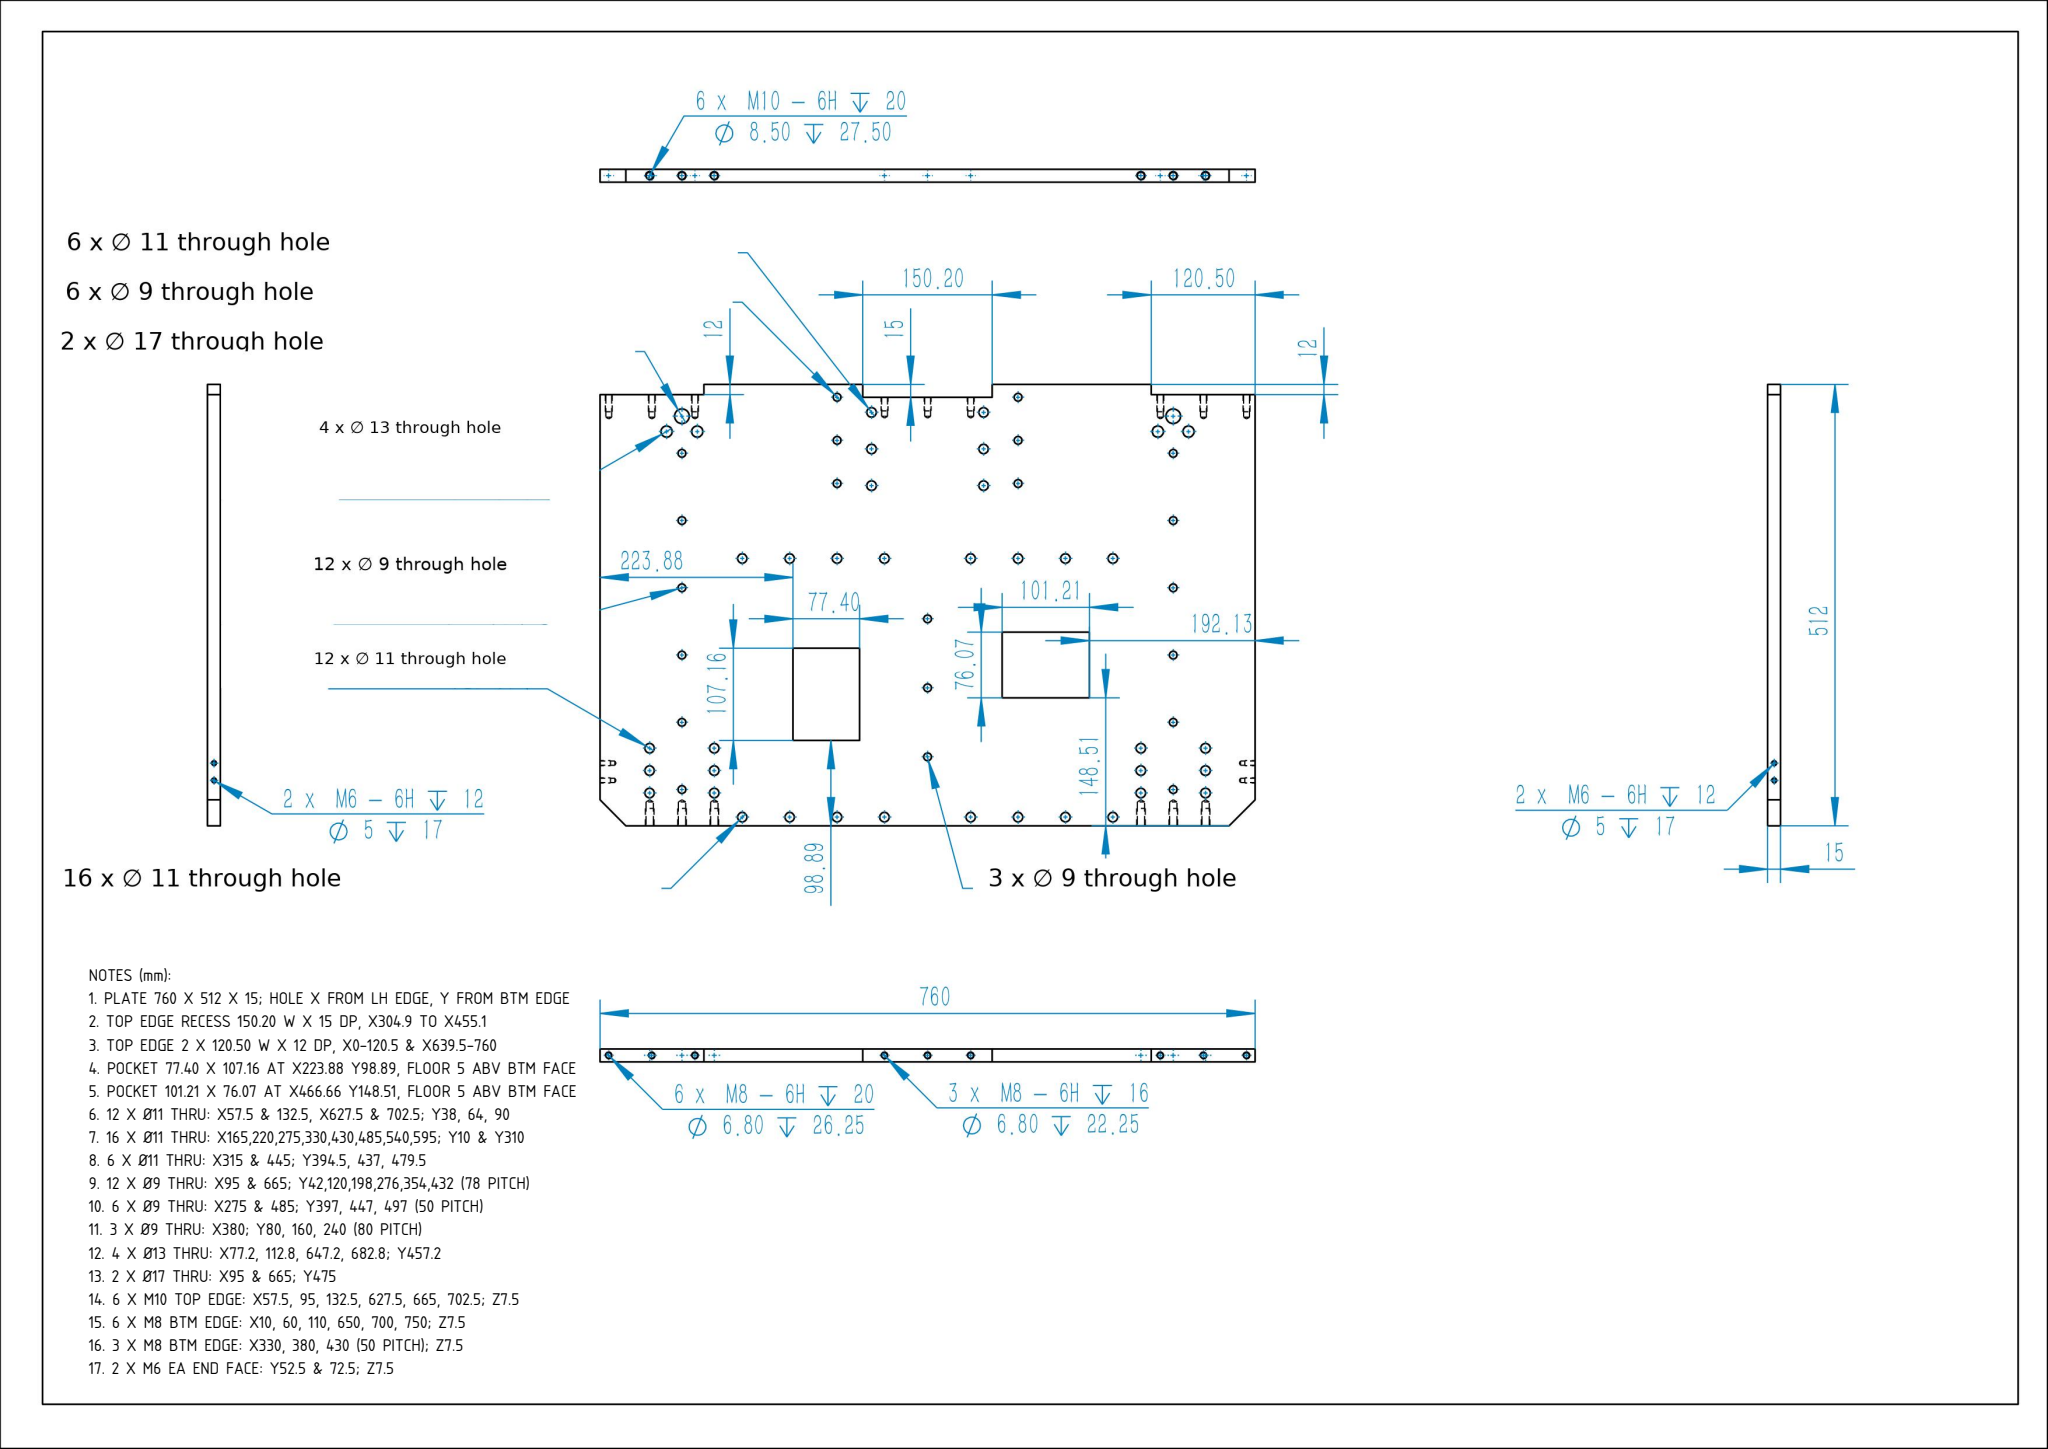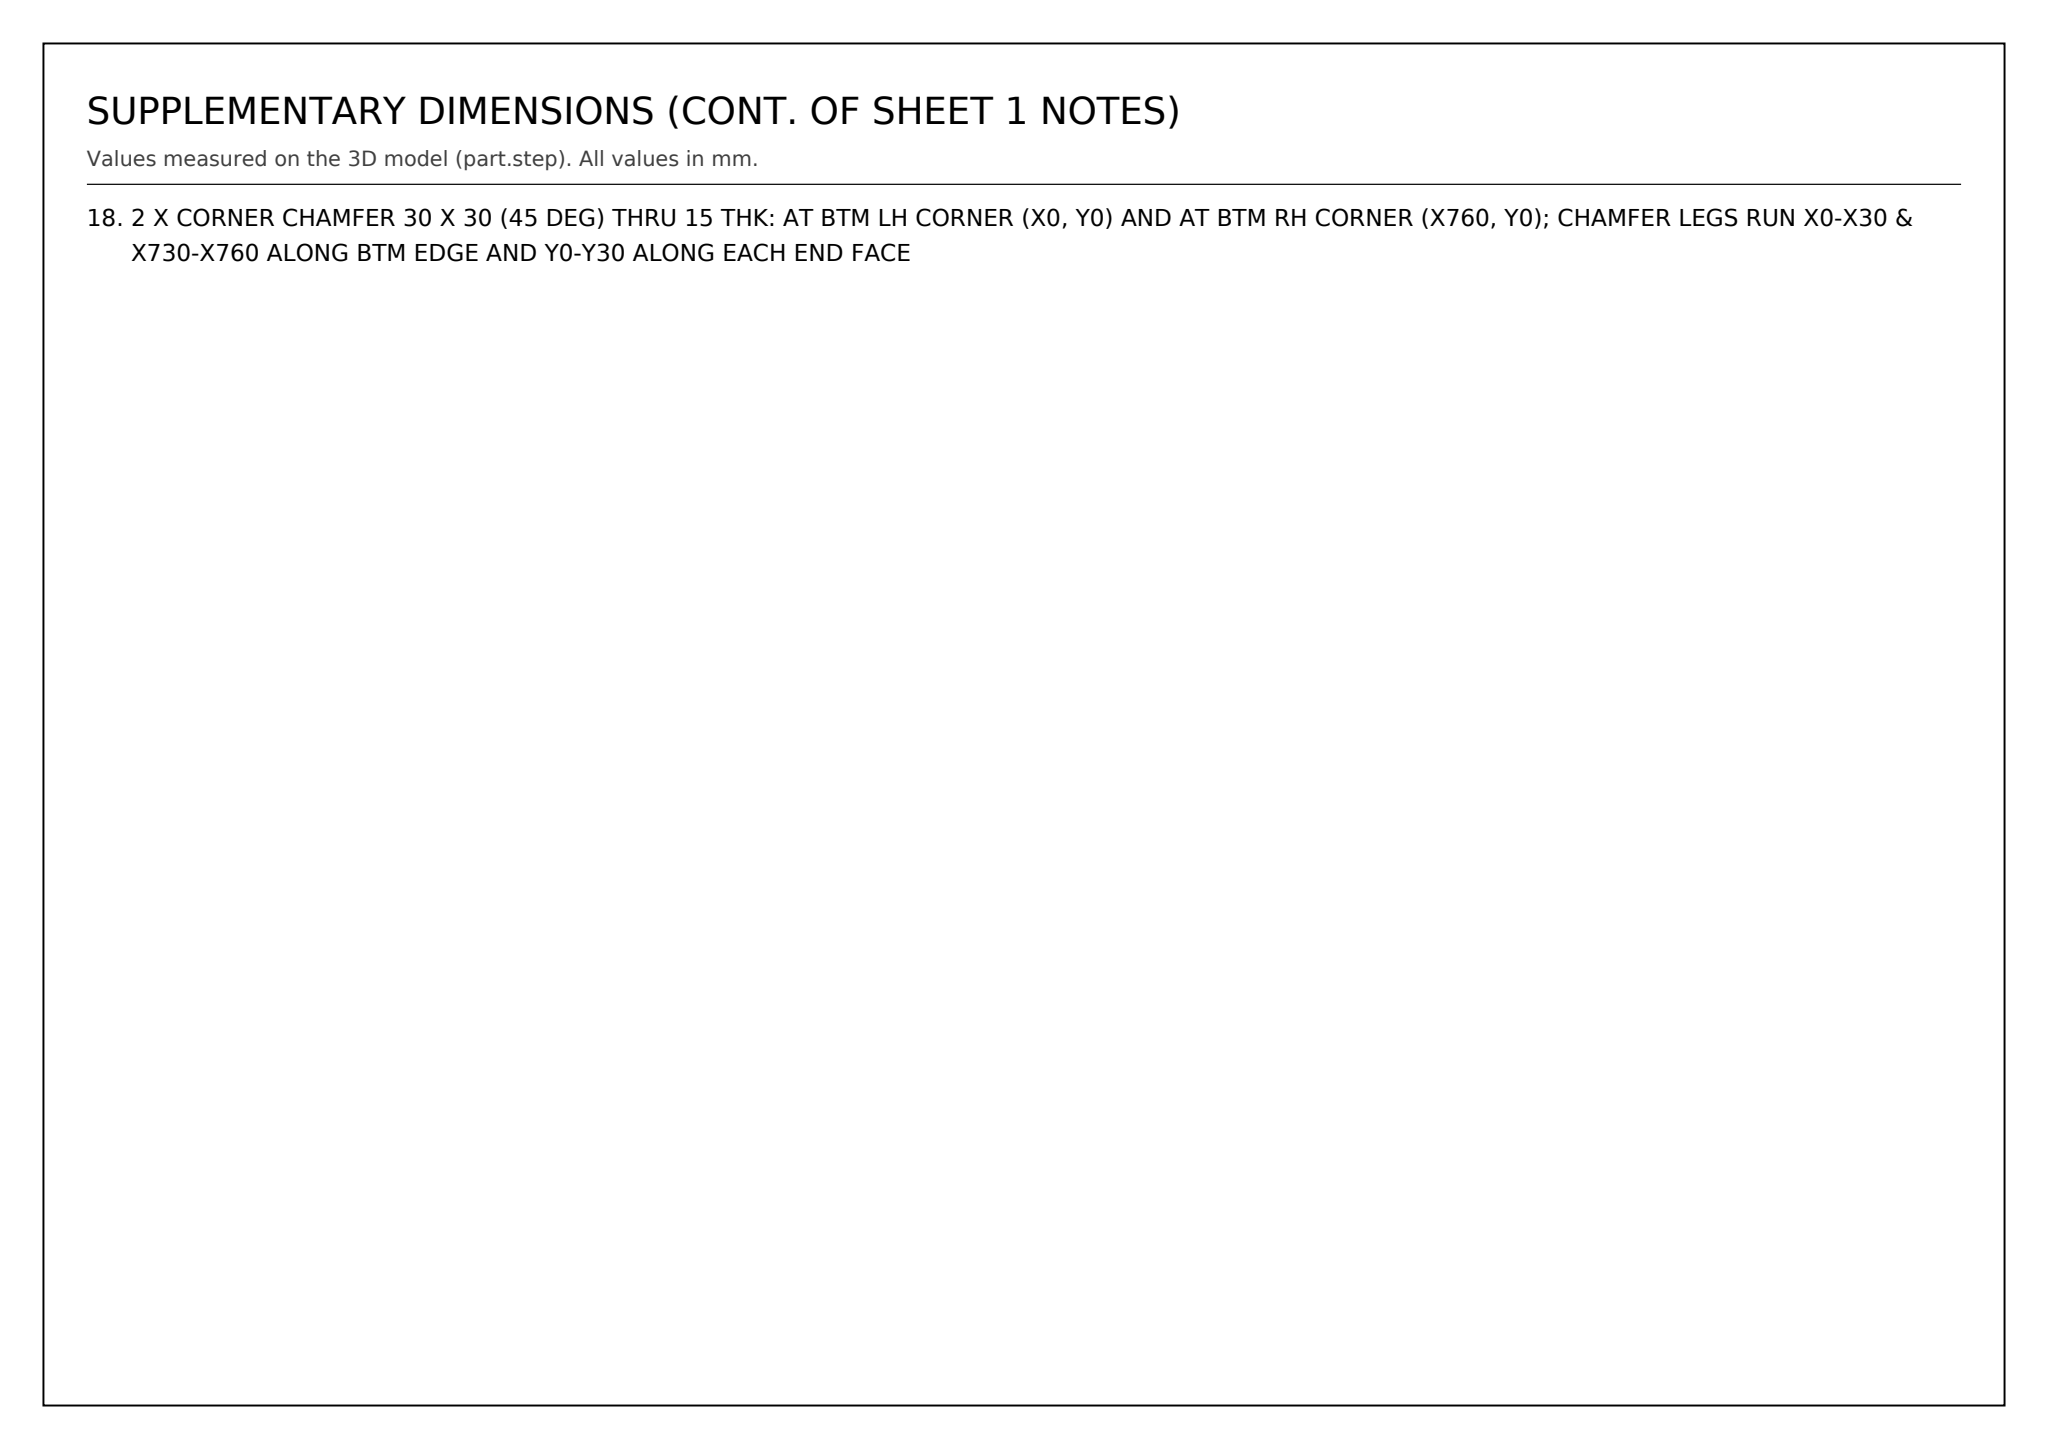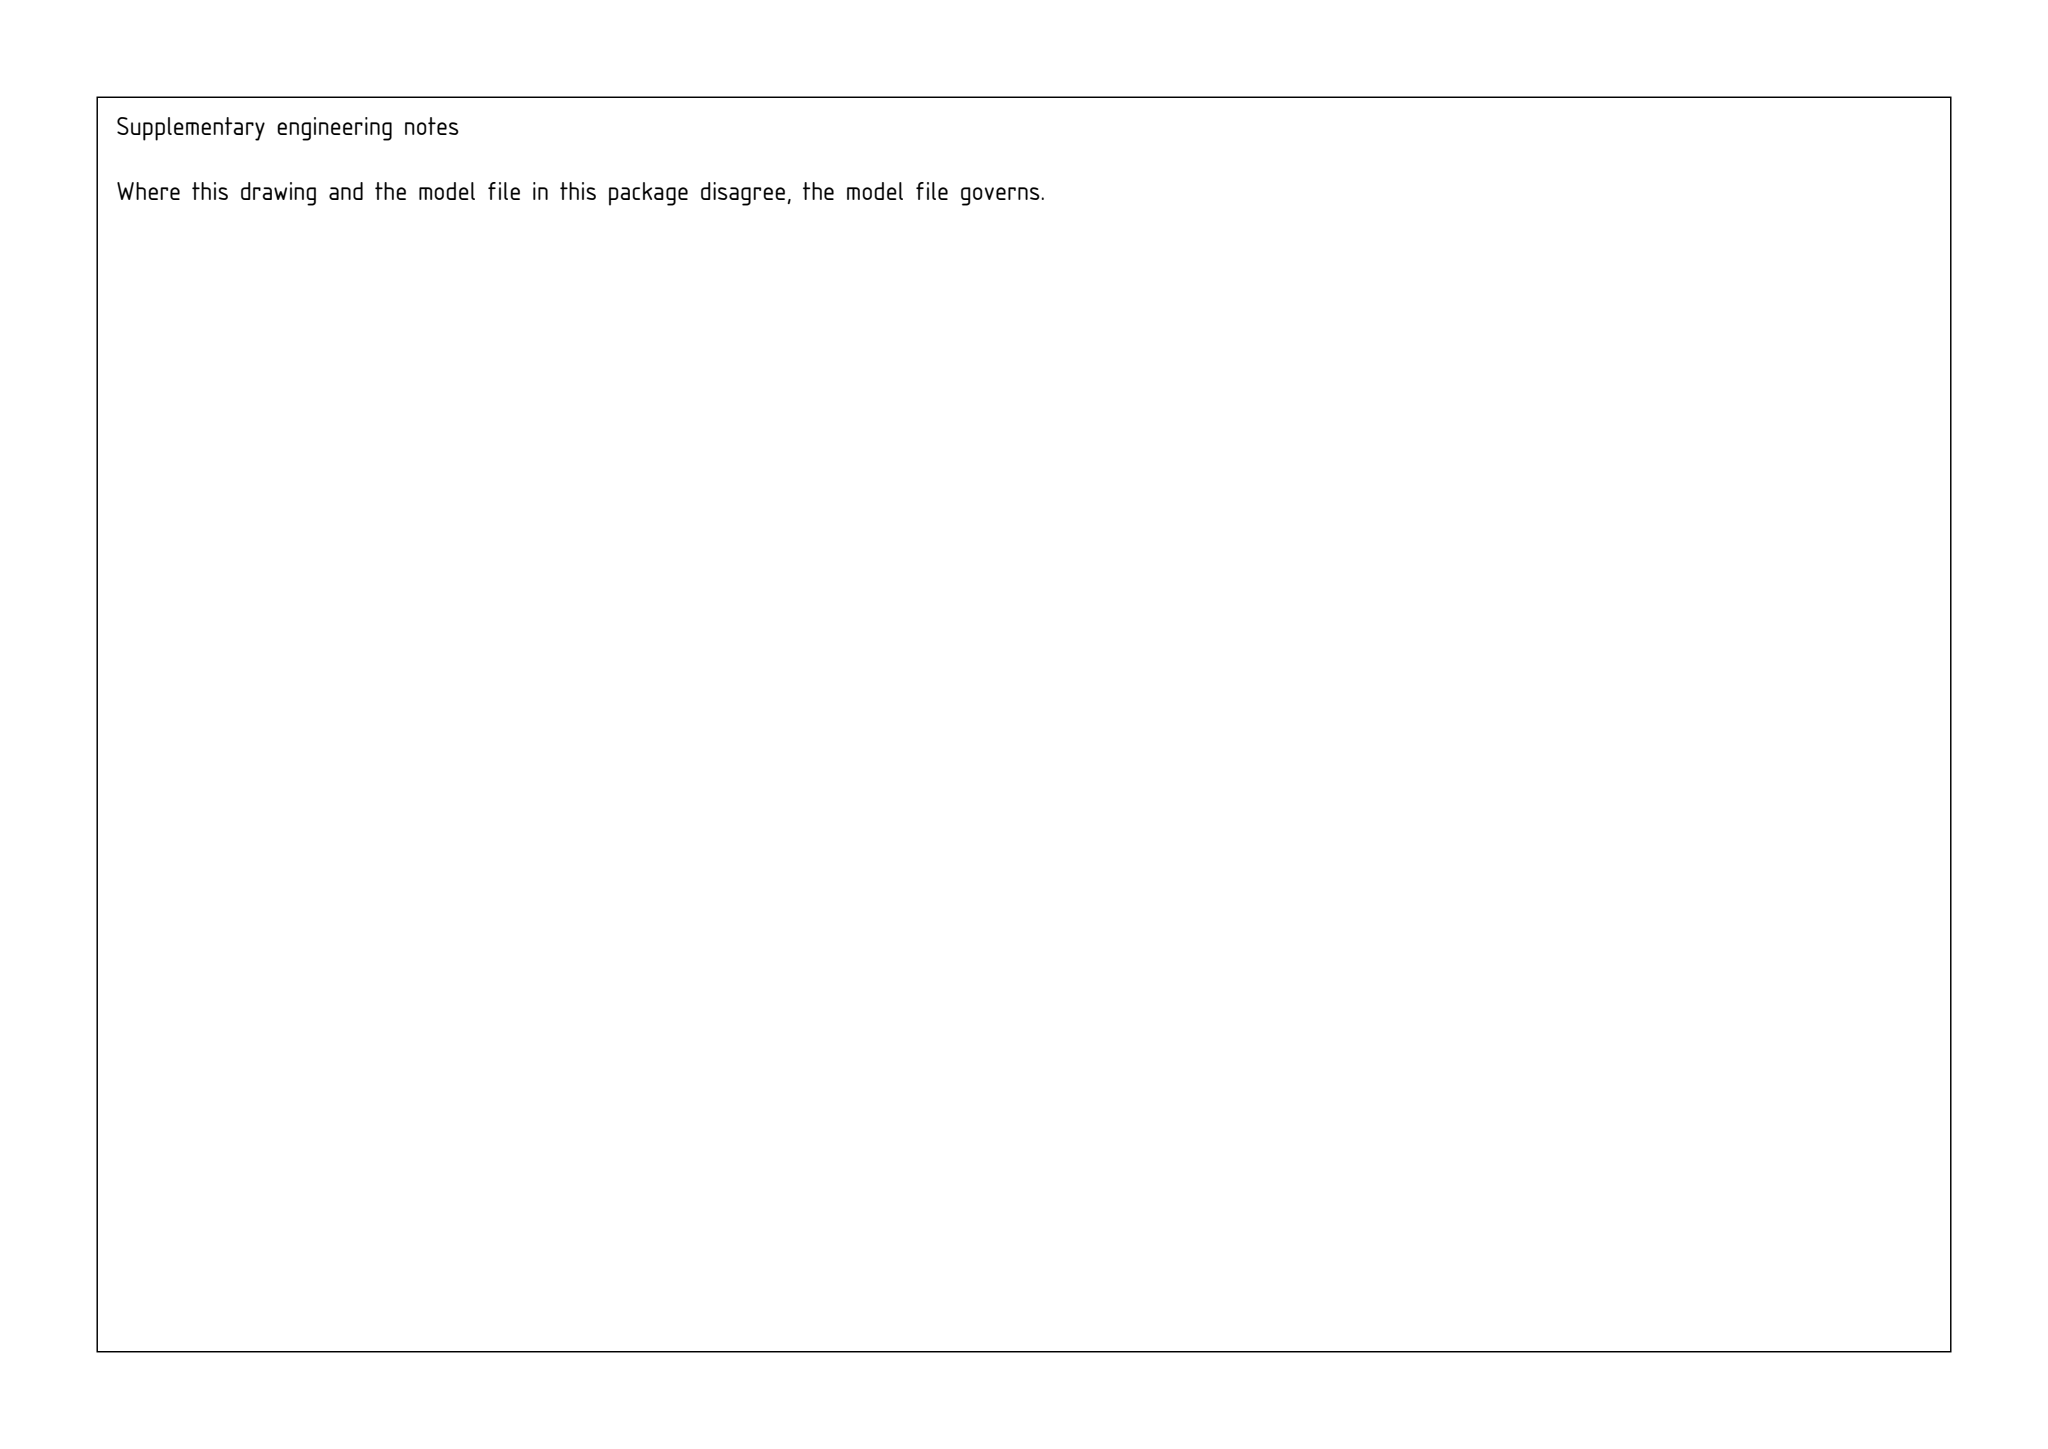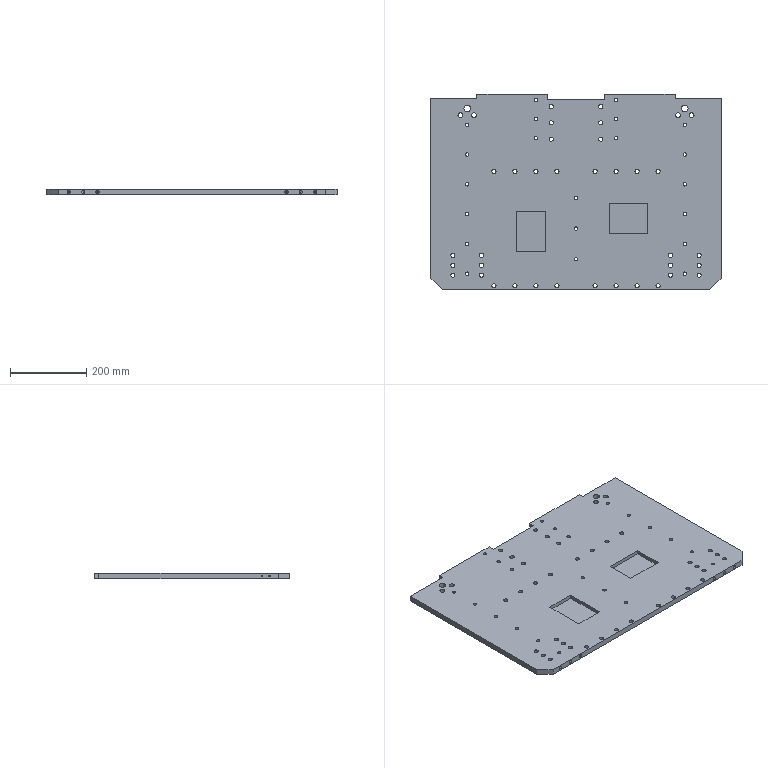Part | SolidWorks | mm | 1 solid | 224 faces | box 760 x 512 x 15 mm | volume 5483517 mm3 | cylinder 160 | cone 38 | plane 26 | commonest cylinder face diameters 11 x68 9 x42 6.8 x18 8.5 x12 5 x8 13 x8 17 x4
Drawing notes:
PLATE 760 X 512 X 15; HOLE X FROM LH EDGE, Y FROM BTM EDGE | from the solid: bbox_xyz [760,512,15], positions from min corner of bbox
TOP EDGE RECESS 150.20 W X 15 DP, X304.9 TO X455.1 | from the solid: x planes 304.9/455.1, y plane 497 vs 512 edge
TOP EDGE 2 X 120.50 W X 12 DP, X0-120.5 & X639.5-760 | from the solid: x planes 120.5/639.5, y planes 500 (2 faces) vs 512
POCKET 77.40 X 107.16 AT X223.88 Y98.89, FLOOR 5 ABV BTM FACE | from the solid: x planes 223.88/301.28, y planes 98.89/206.06, z plane 5
POCKET 101.21 X 76.07 AT X466.66 Y148.51, FLOOR 5 ABV BTM FACE | from the solid: x planes 466.66/567.87, y planes 148.51/224.58, z plane 5
12 X Ø11 THRU: X57.5 & 132.5, X627.5 & 702.5; Y38, 64, 90 | from the solid: Ø11 cyls at (57.5/132.5/627.5/702.5, 38/64/90), L=15 thru
16 X Ø11 THRU: X165,220,275,330,430,485,540,595; Y10 & Y310 | from the solid: Ø11 cyls at those X with y=10 and y=310, L=15 thru
6 X Ø11 THRU: X315 & 445; Y394.5, 437, 479.5 | from the solid: Ø11 cyls (315/445, 394.5/437/479.5), L=15 thru
12 X Ø9 THRU: X95 & 665; Y42,120,198,276,354,432 (78 PITCH) | from the solid: Ø9 cyls at x=95 & 665, y=42..432 step 78, L=15 thru
6 X Ø9 THRU: X275 & 485; Y397, 447, 497 (50 PITCH) | from the solid: Ø9 cyls at x=275 & 485, y=397/447/497, L=15 thru
3 X Ø9 THRU: X380; Y80, 160, 240 (80 PITCH) | from the solid: Ø9 cyls at x=380, y=80/160/240, L=15 thru
4 X Ø13 THRU: X77.2, 112.8, 647.2, 682.8; Y457.2 | from the solid: Ø13 cyls at y=457.2, x=77.2/112.8/647.2/682.8, L=15 thru
2 X Ø17 THRU: X95 & 665; Y475 | from the solid: Ø17 cyls at (95,475) and (665,475), L=15 thru
6 X M10 TOP EDGE: X57.5, 95, 132.5, 627.5, 665, 702.5; Z7.5 | from the solid: Ø8.5 y-axis cyls at those X, z=7.5, L=27.5
6 X M8 BTM EDGE: X10, 60, 110, 650, 700, 750; Z7.5 | from the solid: Ø6.8 y-axis cyls L=26.25 at x=10/60/110/650/700/750, z=7.5
3 X M8 BTM EDGE: X330, 380, 430 (50 PITCH); Z7.5 | from the solid: Ø6.8 y-axis cyls L=22.25 at x=330/380/430, z=7.5
2 X M6 EA END FACE: Y52.5 & 72.5; Z7.5 | from the solid: Ø5 x-axis cyls at y=52.5 & 72.5, z=7.5, L=17
2 X CORNER CHAMFER 30 X 30 (45 DEG) THRU 15 THK: AT BTM LH CORNER (X0, Y0) AND AT BTM RH CORNER (X760, Y0); CHAMFER LEGS RUN X0-X30 & X730-X760 ALONG BTM EDGE AND Y0-Y30 ALONG EACH END FACE | from the solid: inclined_planes: angle_to_xyz_axes [45,45,90], bbox_from [0,0,0] size [30,30,15] and bbox_from [730,0,0] size [30,30,15]; axis_planes y=0 extent x[30,730], x=0 and x=760 extent y[30,500]